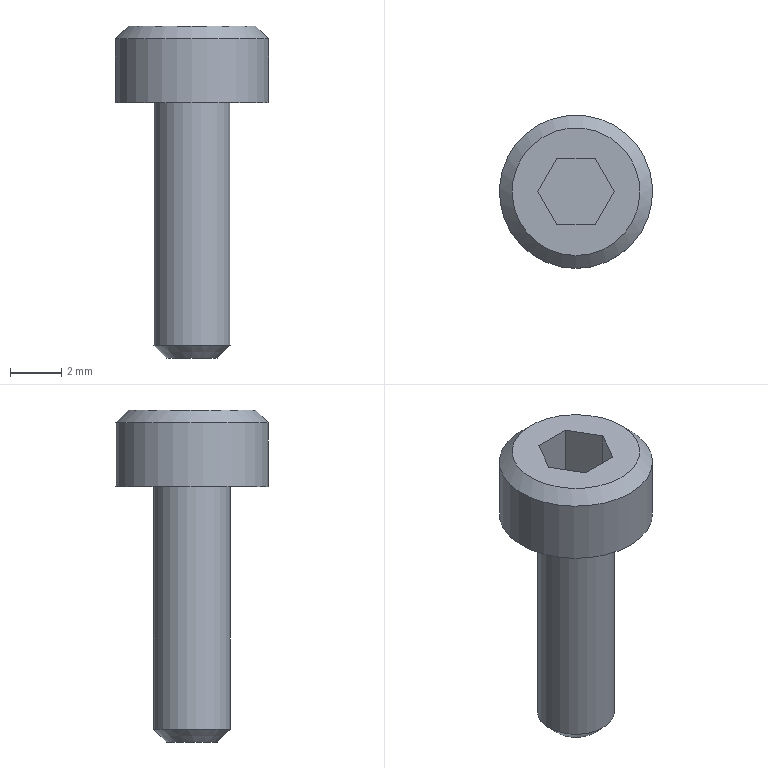Component | NX | SCREW_2 | 1 solid | 14 faces | box 6 x 6 x 13 mm | volume 141 mm3 | plane 10 | cylinder 2 | cone 2 | commonest cylinder face diameters 6 x1 3 x1
STEP:
#1=CARTESIAN_POINT('',(0.,0.,0.));
#2=DIRECTION('',(0.,0.,1.));
#3=DIRECTION('',(1.,0.,0.));
#4=AXIS2_PLACEMENT_3D('',#1,#2,#3);
#5=CARTESIAN_POINT('',(-30.505,120.395,118.114));
#6=VERTEX_POINT('',#5);
#7=CARTESIAN_POINT('',(-30.505,122.895,118.114));
#8=DIRECTION('',(0.,0.,1.));
#9=DIRECTION('',(0.,-1.,0.));
#10=AXIS2_PLACEMENT_3D('',#7,#8,#9);
#11=CIRCLE('',#10,2.5);
#12=CARTESIAN_POINT('',(-30.505,122.895,118.114));
#13=DIRECTION('',(0.,0.,1.));
#14=DIRECTION('',(0.,-1.,0.));
#15=AXIS2_PLACEMENT_3D('',#12,#13,#14);
#16=PLANE('',#15);
#17=CARTESIAN_POINT('',(0.,0.));
#18=DIRECTION('',(1.,0.));
#19=AXIS2_PLACEMENT_2D('',#17,#18);
#20=CIRCLE('',#19,2.5);
#21=(GEOMETRIC_REPRESENTATION_CONTEXT(2)PARAMETRIC_REPRESENTATION_CONTEXT()REPRESENTATION_CONTEXT('',''));
#22=DEFINITIONAL_REPRESENTATION('',(#20),#21);
#23=PCURVE('',#16,#22);
#24=CARTESIAN_POINT('',(-30.505,122.895,118.114));
#25=DIRECTION('',(0.,-0.,-1.));
#26=DIRECTION('',(0.,1.,-0.));
#27=AXIS2_PLACEMENT_3D('',#24,#25,#26);
#28=CONICAL_SURFACE('',#27,2.5,0.7854);
#29=CARTESIAN_POINT('',(9.425,0.));
#30=DIRECTION('',(-1.,0.));
#31=VECTOR('',#30,1.);
#32=LINE('',#29,#31);
#33=(GEOMETRIC_REPRESENTATION_CONTEXT(2)PARAMETRIC_REPRESENTATION_CONTEXT()REPRESENTATION_CONTEXT('',''));
#34=DEFINITIONAL_REPRESENTATION('',(#32),#33);
#35=PCURVE('',#28,#34);
#36=SURFACE_CURVE('',#11,(#23,#35),.PCURVE_S1.);
#37=EDGE_CURVE('',#6,#6,#36,.T.);
#38=ORIENTED_EDGE('',*,*,#37,.T.);
#39=EDGE_LOOP('',(#38));
#40=FACE_BOUND('',#39,.T.);
#41=CARTESIAN_POINT('',(-31.255,121.595,118.114));
#42=VERTEX_POINT('',#41);
#43=CARTESIAN_POINT('',(-29.755,121.595,118.114));
#44=VERTEX_POINT('',#43);
#45=CARTESIAN_POINT('',(-31.255,121.595,118.114));
#46=DIRECTION('',(1.,-0.,0.));
#47=VECTOR('',#46,1.);
#48=LINE('',#45,#47);
#49=CARTESIAN_POINT('',(1.299,-0.75));
#50=DIRECTION('',(0.,1.));
#51=VECTOR('',#50,1.);
#52=LINE('',#49,#51);
#53=(GEOMETRIC_REPRESENTATION_CONTEXT(2)PARAMETRIC_REPRESENTATION_CONTEXT()REPRESENTATION_CONTEXT('',''));
#54=DEFINITIONAL_REPRESENTATION('',(#52),#53);
#55=PCURVE('',#16,#54);
#56=CARTESIAN_POINT('',(-31.255,121.595,116.114));
#57=DIRECTION('',(-0.,-1.,0.));
#58=DIRECTION('',(-1.,0.,-0.));
#59=AXIS2_PLACEMENT_3D('',#56,#57,#58);
#60=PLANE('',#59);
#61=CARTESIAN_POINT('',(-0.,-2.));
#62=DIRECTION('',(-1.,-0.));
#63=VECTOR('',#62,1.);
#64=LINE('',#61,#63);
#65=(GEOMETRIC_REPRESENTATION_CONTEXT(2)PARAMETRIC_REPRESENTATION_CONTEXT()REPRESENTATION_CONTEXT('',''));
#66=DEFINITIONAL_REPRESENTATION('',(#64),#65);
#67=PCURVE('',#60,#66);
#68=SURFACE_CURVE('',#48,(#55,#67),.PCURVE_S1.);
#69=EDGE_CURVE('',#42,#44,#68,.T.);
#70=ORIENTED_EDGE('',*,*,#69,.F.);
#71=CARTESIAN_POINT('',(-32.005,122.895,118.114));
#72=VERTEX_POINT('',#71);
#73=CARTESIAN_POINT('',(-32.005,122.895,118.114));
#74=DIRECTION('',(0.5,-0.866,0.));
#75=VECTOR('',#74,1.);
#76=LINE('',#73,#75);
#77=CARTESIAN_POINT('',(0.,-1.5));
#78=DIRECTION('',(0.866,0.5));
#79=VECTOR('',#78,1.);
#80=LINE('',#77,#79);
#81=(GEOMETRIC_REPRESENTATION_CONTEXT(2)PARAMETRIC_REPRESENTATION_CONTEXT()REPRESENTATION_CONTEXT('',''));
#82=DEFINITIONAL_REPRESENTATION('',(#80),#81);
#83=PCURVE('',#16,#82);
#84=CARTESIAN_POINT('',(-32.005,122.895,116.114));
#85=DIRECTION('',(-0.866,-0.5,0.));
#86=DIRECTION('',(-0.5,0.866,0.));
#87=AXIS2_PLACEMENT_3D('',#84,#85,#86);
#88=PLANE('',#87);
#89=CARTESIAN_POINT('',(0.,-2.));
#90=DIRECTION('',(-1.,-0.));
#91=VECTOR('',#90,1.);
#92=LINE('',#89,#91);
#93=(GEOMETRIC_REPRESENTATION_CONTEXT(2)PARAMETRIC_REPRESENTATION_CONTEXT()REPRESENTATION_CONTEXT('',''));
#94=DEFINITIONAL_REPRESENTATION('',(#92),#93);
#95=PCURVE('',#88,#94);
#96=SURFACE_CURVE('',#76,(#83,#95),.PCURVE_S1.);
#97=EDGE_CURVE('',#72,#42,#96,.T.);
#98=ORIENTED_EDGE('',*,*,#97,.F.);
#99=CARTESIAN_POINT('',(-31.255,124.194,118.114));
#100=VERTEX_POINT('',#99);
#101=CARTESIAN_POINT('',(-31.255,124.194,118.114));
#102=DIRECTION('',(-0.5,-0.866,0.));
#103=VECTOR('',#102,1.);
#104=LINE('',#101,#103);
#105=CARTESIAN_POINT('',(-1.299,-0.75));
#106=DIRECTION('',(0.866,-0.5));
#107=VECTOR('',#106,1.);
#108=LINE('',#105,#107);
#109=(GEOMETRIC_REPRESENTATION_CONTEXT(2)PARAMETRIC_REPRESENTATION_CONTEXT()REPRESENTATION_CONTEXT('',''));
#110=DEFINITIONAL_REPRESENTATION('',(#108),#109);
#111=PCURVE('',#16,#110);
#112=CARTESIAN_POINT('',(-31.255,124.194,116.114));
#113=DIRECTION('',(-0.866,0.5,-0.));
#114=DIRECTION('',(0.5,0.866,0.));
#115=AXIS2_PLACEMENT_3D('',#112,#113,#114);
#116=PLANE('',#115);
#117=CARTESIAN_POINT('',(0.,-2.));
#118=DIRECTION('',(-1.,-0.));
#119=VECTOR('',#118,1.);
#120=LINE('',#117,#119);
#121=(GEOMETRIC_REPRESENTATION_CONTEXT(2)PARAMETRIC_REPRESENTATION_CONTEXT()REPRESENTATION_CONTEXT('',''));
#122=DEFINITIONAL_REPRESENTATION('',(#120),#121);
#123=PCURVE('',#116,#122);
#124=SURFACE_CURVE('',#104,(#111,#123),.PCURVE_S1.);
#125=EDGE_CURVE('',#100,#72,#124,.T.);
#126=ORIENTED_EDGE('',*,*,#125,.F.);
#127=CARTESIAN_POINT('',(-29.755,124.194,118.114));
#128=VERTEX_POINT('',#127);
#129=CARTESIAN_POINT('',(-29.755,124.194,118.114));
#130=DIRECTION('',(-1.,0.,-0.));
#131=VECTOR('',#130,1.);
#132=LINE('',#129,#131);
#133=CARTESIAN_POINT('',(-1.299,0.75));
#134=DIRECTION('',(-0.,-1.));
#135=VECTOR('',#134,1.);
#136=LINE('',#133,#135);
#137=(GEOMETRIC_REPRESENTATION_CONTEXT(2)PARAMETRIC_REPRESENTATION_CONTEXT()REPRESENTATION_CONTEXT('',''));
#138=DEFINITIONAL_REPRESENTATION('',(#136),#137);
#139=PCURVE('',#16,#138);
#140=CARTESIAN_POINT('',(-29.755,124.194,116.114));
#141=DIRECTION('',(0.,1.,-0.));
#142=DIRECTION('',(1.,-0.,0.));
#143=AXIS2_PLACEMENT_3D('',#140,#141,#142);
#144=PLANE('',#143);
#145=CARTESIAN_POINT('',(0.,-2.));
#146=DIRECTION('',(-1.,0.));
#147=VECTOR('',#146,1.);
#148=LINE('',#145,#147);
#149=(GEOMETRIC_REPRESENTATION_CONTEXT(2)PARAMETRIC_REPRESENTATION_CONTEXT()REPRESENTATION_CONTEXT('',''));
#150=DEFINITIONAL_REPRESENTATION('',(#148),#149);
#151=PCURVE('',#144,#150);
#152=SURFACE_CURVE('',#132,(#139,#151),.PCURVE_S1.);
#153=EDGE_CURVE('',#128,#100,#152,.T.);
#154=ORIENTED_EDGE('',*,*,#153,.F.);
#155=CARTESIAN_POINT('',(-29.005,122.895,118.114));
#156=VERTEX_POINT('',#155);
#157=CARTESIAN_POINT('',(-29.005,122.895,118.114));
#158=DIRECTION('',(-0.5,0.866,-0.));
#159=VECTOR('',#158,1.);
#160=LINE('',#157,#159);
#161=CARTESIAN_POINT('',(0.,1.5));
#162=DIRECTION('',(-0.866,-0.5));
#163=VECTOR('',#162,1.);
#164=LINE('',#161,#163);
#165=(GEOMETRIC_REPRESENTATION_CONTEXT(2)PARAMETRIC_REPRESENTATION_CONTEXT()REPRESENTATION_CONTEXT('',''));
#166=DEFINITIONAL_REPRESENTATION('',(#164),#165);
#167=PCURVE('',#16,#166);
#168=CARTESIAN_POINT('',(-29.005,122.895,116.114));
#169=DIRECTION('',(0.866,0.5,-0.));
#170=DIRECTION('',(0.5,-0.866,-0.));
#171=AXIS2_PLACEMENT_3D('',#168,#169,#170);
#172=PLANE('',#171);
#173=CARTESIAN_POINT('',(-0.,-2.));
#174=DIRECTION('',(-1.,0.));
#175=VECTOR('',#174,1.);
#176=LINE('',#173,#175);
#177=(GEOMETRIC_REPRESENTATION_CONTEXT(2)PARAMETRIC_REPRESENTATION_CONTEXT()REPRESENTATION_CONTEXT('',''));
#178=DEFINITIONAL_REPRESENTATION('',(#176),#177);
#179=PCURVE('',#172,#178);
#180=SURFACE_CURVE('',#160,(#167,#179),.PCURVE_S1.);
#181=EDGE_CURVE('',#156,#128,#180,.T.);
#182=ORIENTED_EDGE('',*,*,#181,.F.);
#183=CARTESIAN_POINT('',(-29.755,121.595,118.114));
#184=DIRECTION('',(0.5,0.866,-0.));
#185=VECTOR('',#184,1.);
#186=LINE('',#183,#185);
#187=CARTESIAN_POINT('',(1.299,0.75));
#188=DIRECTION('',(-0.866,0.5));
#189=VECTOR('',#188,1.);
#190=LINE('',#187,#189);
#191=(GEOMETRIC_REPRESENTATION_CONTEXT(2)PARAMETRIC_REPRESENTATION_CONTEXT()REPRESENTATION_CONTEXT('',''));
#192=DEFINITIONAL_REPRESENTATION('',(#190),#191);
#193=PCURVE('',#16,#192);
#194=CARTESIAN_POINT('',(-29.755,121.595,116.114));
#195=DIRECTION('',(0.866,-0.5,0.));
#196=DIRECTION('',(-0.5,-0.866,0.));
#197=AXIS2_PLACEMENT_3D('',#194,#195,#196);
#198=PLANE('',#197);
#199=CARTESIAN_POINT('',(0.,-2.));
#200=DIRECTION('',(-1.,0.));
#201=VECTOR('',#200,1.);
#202=LINE('',#199,#201);
#203=(GEOMETRIC_REPRESENTATION_CONTEXT(2)PARAMETRIC_REPRESENTATION_CONTEXT()REPRESENTATION_CONTEXT('',''));
#204=DEFINITIONAL_REPRESENTATION('',(#202),#203);
#205=PCURVE('',#198,#204);
#206=SURFACE_CURVE('',#186,(#193,#205),.PCURVE_S1.);
#207=EDGE_CURVE('',#44,#156,#206,.T.);
#208=ORIENTED_EDGE('',*,*,#207,.F.);
#209=EDGE_LOOP('',(#70,#98,#126,#154,#182,#208));
#210=FACE_BOUND('',#209,.T.);
#211=ADVANCED_FACE('',(#40,#210),#16,.T.);
#212=CARTESIAN_POINT('',(-30.505,119.895,117.614));
#213=VERTEX_POINT('',#212);
#214=CARTESIAN_POINT('',(-30.505,122.895,117.614));
#215=DIRECTION('',(0.,-0.,-1.));
#216=DIRECTION('',(0.,-1.,0.));
#217=AXIS2_PLACEMENT_3D('',#214,#215,#216);
#218=CIRCLE('',#217,3.);
#219=CARTESIAN_POINT('',(-30.505,122.895,105.114));
#220=DIRECTION('',(0.,0.,1.));
#221=DIRECTION('',(0.,-1.,0.));
#222=AXIS2_PLACEMENT_3D('',#219,#220,#221);
#223=CYLINDRICAL_SURFACE('',#222,3.);
#224=CARTESIAN_POINT('',(6.283,12.5));
#225=DIRECTION('',(-1.,0.));
#226=VECTOR('',#225,1.);
#227=LINE('',#224,#226);
#228=(GEOMETRIC_REPRESENTATION_CONTEXT(2)PARAMETRIC_REPRESENTATION_CONTEXT()REPRESENTATION_CONTEXT('',''));
#229=DEFINITIONAL_REPRESENTATION('',(#227),#228);
#230=PCURVE('',#223,#229);
#231=CARTESIAN_POINT('',(3.142,0.5));
#232=DIRECTION('',(1.,0.));
#233=VECTOR('',#232,1.);
#234=LINE('',#231,#233);
#235=(GEOMETRIC_REPRESENTATION_CONTEXT(2)PARAMETRIC_REPRESENTATION_CONTEXT()REPRESENTATION_CONTEXT('',''));
#236=DEFINITIONAL_REPRESENTATION('',(#234),#235);
#237=PCURVE('',#28,#236);
#238=SURFACE_CURVE('',#218,(#230,#237),.PCURVE_S1.);
#239=EDGE_CURVE('',#213,#213,#238,.T.);
#240=ORIENTED_EDGE('',*,*,#239,.T.);
#241=CARTESIAN_POINT('',(-30.505,119.895,115.114));
#242=VERTEX_POINT('',#241);
#243=CARTESIAN_POINT('',(-30.505,119.895,115.114));
#244=CARTESIAN_POINT('',(-30.505,119.895,117.614));
#245=B_SPLINE_CURVE_WITH_KNOTS('',1,(#243,#244),.UNSPECIFIED.,.F.,.F.,(2,2),(10.,12.5),.PIECEWISE_BEZIER_KNOTS.);
#246=CARTESIAN_POINT('',(0.,0.));
#247=DIRECTION('',(0.,1.));
#248=VECTOR('',#247,1.);
#249=LINE('',#246,#248);
#250=(GEOMETRIC_REPRESENTATION_CONTEXT(2)PARAMETRIC_REPRESENTATION_CONTEXT()REPRESENTATION_CONTEXT('',''));
#251=DEFINITIONAL_REPRESENTATION('',(#249),#250);
#252=PCURVE('',#223,#251);
#253=CARTESIAN_POINT('',(6.283,0.));
#254=DIRECTION('',(0.,1.));
#255=VECTOR('',#254,1.);
#256=LINE('',#253,#255);
#257=(GEOMETRIC_REPRESENTATION_CONTEXT(2)PARAMETRIC_REPRESENTATION_CONTEXT()REPRESENTATION_CONTEXT('',''));
#258=DEFINITIONAL_REPRESENTATION('',(#256),#257);
#259=PCURVE('',#223,#258);
#260=SEAM_CURVE('',#245,(#252,#259),.PCURVE_S1.);
#261=EDGE_CURVE('',#242,#213,#260,.T.);
#262=ORIENTED_EDGE('',*,*,#261,.F.);
#263=CARTESIAN_POINT('',(-30.505,122.895,115.114));
#264=DIRECTION('',(0.,0.,1.));
#265=DIRECTION('',(0.,-1.,0.));
#266=AXIS2_PLACEMENT_3D('',#263,#264,#265);
#267=CIRCLE('',#266,3.);
#268=CARTESIAN_POINT('',(0.,10.));
#269=DIRECTION('',(1.,0.));
#270=VECTOR('',#269,1.);
#271=LINE('',#268,#270);
#272=(GEOMETRIC_REPRESENTATION_CONTEXT(2)PARAMETRIC_REPRESENTATION_CONTEXT()REPRESENTATION_CONTEXT('',''));
#273=DEFINITIONAL_REPRESENTATION('',(#271),#272);
#274=PCURVE('',#223,#273);
#275=CARTESIAN_POINT('',(-30.505,119.895,115.114));
#276=DIRECTION('',(0.,-0.,-1.));
#277=DIRECTION('',(0.,1.,-0.));
#278=AXIS2_PLACEMENT_3D('',#275,#276,#277);
#279=PLANE('',#278);
#280=CARTESIAN_POINT('',(-0.,0.));
#281=CARTESIAN_POINT('',(-0.,5.196));
#282=CARTESIAN_POINT('',(4.5,2.598));
#283=CARTESIAN_POINT('',(9.,0.));
#284=CARTESIAN_POINT('',(4.5,-2.598));
#285=CARTESIAN_POINT('',(-0.,-5.196));
#286=CARTESIAN_POINT('',(-0.,0.));
#287=(BOUNDED_CURVE()B_SPLINE_CURVE(2,(#280,#281,#282,#283,#284,#285,#286),.UNSPECIFIED.,.T.,.F.)B_SPLINE_CURVE_WITH_KNOTS((1,2,2,2,2,1),(-2.094,0.,2.094,4.189,6.283,8.378),.UNSPECIFIED.)CURVE()GEOMETRIC_REPRESENTATION_ITEM()RATIONAL_B_SPLINE_CURVE((1.,0.5,1.,0.5,1.,0.5,1.))REPRESENTATION_ITEM(''));
#288=(GEOMETRIC_REPRESENTATION_CONTEXT(2)PARAMETRIC_REPRESENTATION_CONTEXT()REPRESENTATION_CONTEXT('',''));
#289=DEFINITIONAL_REPRESENTATION('',(#287),#288);
#290=PCURVE('',#279,#289);
#291=SURFACE_CURVE('',#267,(#274,#290),.PCURVE_S1.);
#292=EDGE_CURVE('',#242,#242,#291,.T.);
#293=ORIENTED_EDGE('',*,*,#292,.T.);
#294=ORIENTED_EDGE('',*,*,#261,.T.);
#295=EDGE_LOOP('',(#240,#262,#293,#294));
#296=FACE_BOUND('',#295,.T.);
#297=ADVANCED_FACE('',(#296),#223,.T.);
#298=CARTESIAN_POINT('',(-30.505,121.395,115.114));
#299=VERTEX_POINT('',#298);
#300=CARTESIAN_POINT('',(-30.505,122.895,115.114));
#301=DIRECTION('',(0.,0.,1.));
#302=DIRECTION('',(0.,-1.,0.));
#303=AXIS2_PLACEMENT_3D('',#300,#301,#302);
#304=CIRCLE('',#303,1.5);
#305=CARTESIAN_POINT('',(1.5,0.));
#306=CARTESIAN_POINT('',(1.5,2.598));
#307=CARTESIAN_POINT('',(3.75,1.299));
#308=CARTESIAN_POINT('',(6.,0.));
#309=CARTESIAN_POINT('',(3.75,-1.299));
#310=CARTESIAN_POINT('',(1.5,-2.598));
#311=CARTESIAN_POINT('',(1.5,0.));
#312=(BOUNDED_CURVE()B_SPLINE_CURVE(2,(#305,#306,#307,#308,#309,#310,#311),.UNSPECIFIED.,.T.,.F.)B_SPLINE_CURVE_WITH_KNOTS((1,2,2,2,2,1),(-2.094,0.,2.094,4.189,6.283,8.378),.UNSPECIFIED.)CURVE()GEOMETRIC_REPRESENTATION_ITEM()RATIONAL_B_SPLINE_CURVE((1.,0.5,1.,0.5,1.,0.5,1.))REPRESENTATION_ITEM(''));
#313=(GEOMETRIC_REPRESENTATION_CONTEXT(2)PARAMETRIC_REPRESENTATION_CONTEXT()REPRESENTATION_CONTEXT('',''));
#314=DEFINITIONAL_REPRESENTATION('',(#312),#313);
#315=PCURVE('',#279,#314);
#316=CARTESIAN_POINT('',(-30.505,122.895,105.114));
#317=DIRECTION('',(0.,0.,1.));
#318=DIRECTION('',(0.,-1.,0.));
#319=AXIS2_PLACEMENT_3D('',#316,#317,#318);
#320=CYLINDRICAL_SURFACE('',#319,1.5);
#321=CARTESIAN_POINT('',(0.,10.));
#322=DIRECTION('',(1.,0.));
#323=VECTOR('',#322,1.);
#324=LINE('',#321,#323);
#325=(GEOMETRIC_REPRESENTATION_CONTEXT(2)PARAMETRIC_REPRESENTATION_CONTEXT()REPRESENTATION_CONTEXT('',''));
#326=DEFINITIONAL_REPRESENTATION('',(#324),#325);
#327=PCURVE('',#320,#326);
#328=SURFACE_CURVE('',#304,(#315,#327),.PCURVE_S1.);
#329=EDGE_CURVE('',#299,#299,#328,.T.);
#330=ORIENTED_EDGE('',*,*,#329,.T.);
#331=EDGE_LOOP('',(#330));
#332=FACE_BOUND('',#331,.T.);
#333=ORIENTED_EDGE('',*,*,#292,.F.);
#334=EDGE_LOOP('',(#333));
#335=FACE_BOUND('',#334,.T.);
#336=ADVANCED_FACE('',(#332,#335),#279,.T.);
#337=CARTESIAN_POINT('',(-30.505,124.395,105.614));
#338=VERTEX_POINT('',#337);
#339=CARTESIAN_POINT('',(-30.505,121.395,105.614));
#340=VERTEX_POINT('',#339);
#341=CARTESIAN_POINT('',(-30.505,122.895,105.614));
#342=DIRECTION('',(0.,0.,1.));
#343=DIRECTION('',(0.,1.,-0.));
#344=AXIS2_PLACEMENT_3D('',#341,#342,#343);
#345=CIRCLE('',#344,1.5);
#346=CARTESIAN_POINT('',(3.142,0.5));
#347=DIRECTION('',(1.,0.));
#348=VECTOR('',#347,1.);
#349=LINE('',#346,#348);
#350=(GEOMETRIC_REPRESENTATION_CONTEXT(2)PARAMETRIC_REPRESENTATION_CONTEXT()REPRESENTATION_CONTEXT('',''));
#351=DEFINITIONAL_REPRESENTATION('',(#349),#350);
#352=PCURVE('',#320,#351);
#353=CARTESIAN_POINT('',(-30.505,122.895,105.614));
#354=DIRECTION('',(0.,0.,1.));
#355=DIRECTION('',(0.,-1.,0.));
#356=AXIS2_PLACEMENT_3D('',#353,#354,#355);
#357=CONICAL_SURFACE('',#356,1.5,0.7854);
#358=CARTESIAN_POINT('',(3.142,0.));
#359=DIRECTION('',(1.,0.));
#360=VECTOR('',#359,1.);
#361=LINE('',#358,#360);
#362=(GEOMETRIC_REPRESENTATION_CONTEXT(2)PARAMETRIC_REPRESENTATION_CONTEXT()REPRESENTATION_CONTEXT('',''));
#363=DEFINITIONAL_REPRESENTATION('',(#361),#362);
#364=PCURVE('',#357,#363);
#365=SURFACE_CURVE('',#345,(#352,#364),.PCURVE_S1.);
#366=EDGE_CURVE('',#338,#340,#365,.T.);
#367=ORIENTED_EDGE('',*,*,#366,.T.);
#368=CARTESIAN_POINT('',(-30.505,121.395,105.614));
#369=CARTESIAN_POINT('',(-30.505,121.395,115.114));
#370=B_SPLINE_CURVE_WITH_KNOTS('',1,(#368,#369),.UNSPECIFIED.,.F.,.F.,(2,2),(0.5,10.),.PIECEWISE_BEZIER_KNOTS.);
#371=CARTESIAN_POINT('',(6.283,0.));
#372=DIRECTION('',(0.,1.));
#373=VECTOR('',#372,1.);
#374=LINE('',#371,#373);
#375=(GEOMETRIC_REPRESENTATION_CONTEXT(2)PARAMETRIC_REPRESENTATION_CONTEXT()REPRESENTATION_CONTEXT('',''));
#376=DEFINITIONAL_REPRESENTATION('',(#374),#375);
#377=PCURVE('',#320,#376);
#378=CARTESIAN_POINT('',(0.,0.));
#379=DIRECTION('',(0.,1.));
#380=VECTOR('',#379,1.);
#381=LINE('',#378,#380);
#382=(GEOMETRIC_REPRESENTATION_CONTEXT(2)PARAMETRIC_REPRESENTATION_CONTEXT()REPRESENTATION_CONTEXT('',''));
#383=DEFINITIONAL_REPRESENTATION('',(#381),#382);
#384=PCURVE('',#320,#383);
#385=SEAM_CURVE('',#370,(#377,#384),.PCURVE_S1.);
#386=EDGE_CURVE('',#340,#299,#385,.T.);
#387=ORIENTED_EDGE('',*,*,#386,.T.);
#388=ORIENTED_EDGE('',*,*,#329,.F.);
#389=ORIENTED_EDGE('',*,*,#386,.F.);
#390=CARTESIAN_POINT('',(-30.505,122.895,105.614));
#391=DIRECTION('',(0.,0.,1.));
#392=DIRECTION('',(0.,1.,-0.));
#393=AXIS2_PLACEMENT_3D('',#390,#391,#392);
#394=CIRCLE('',#393,1.5);
#395=CARTESIAN_POINT('',(-3.142,0.5));
#396=DIRECTION('',(1.,0.));
#397=VECTOR('',#396,1.);
#398=LINE('',#395,#397);
#399=(GEOMETRIC_REPRESENTATION_CONTEXT(2)PARAMETRIC_REPRESENTATION_CONTEXT()REPRESENTATION_CONTEXT('',''));
#400=DEFINITIONAL_REPRESENTATION('',(#398),#399);
#401=PCURVE('',#320,#400);
#402=CARTESIAN_POINT('',(3.142,0.));
#403=DIRECTION('',(1.,0.));
#404=VECTOR('',#403,1.);
#405=LINE('',#402,#404);
#406=(GEOMETRIC_REPRESENTATION_CONTEXT(2)PARAMETRIC_REPRESENTATION_CONTEXT()REPRESENTATION_CONTEXT('',''));
#407=DEFINITIONAL_REPRESENTATION('',(#405),#406);
#408=PCURVE('',#357,#407);
#409=SURFACE_CURVE('',#394,(#401,#408),.PCURVE_S1.);
#410=EDGE_CURVE('',#340,#338,#409,.T.);
#411=ORIENTED_EDGE('',*,*,#410,.T.);
#412=EDGE_LOOP('',(#367,#387,#388,#389,#411));
#413=FACE_BOUND('',#412,.T.);
#414=ADVANCED_FACE('',(#413),#320,.T.);
#415=CARTESIAN_POINT('',(-30.505,123.895,105.114));
#416=VERTEX_POINT('',#415);
#417=CARTESIAN_POINT('',(-30.505,122.895,105.114));
#418=DIRECTION('',(0.,-0.,-1.));
#419=DIRECTION('',(0.,1.,-0.));
#420=AXIS2_PLACEMENT_3D('',#417,#418,#419);
#421=CIRCLE('',#420,1.);
#422=CARTESIAN_POINT('',(-30.505,121.395,105.114));
#423=DIRECTION('',(0.,-0.,-1.));
#424=DIRECTION('',(0.,1.,-0.));
#425=AXIS2_PLACEMENT_3D('',#422,#423,#424);
#426=PLANE('',#425);
#427=CARTESIAN_POINT('',(1.5,0.));
#428=DIRECTION('',(1.,0.));
#429=AXIS2_PLACEMENT_2D('',#427,#428);
#430=CIRCLE('',#429,1.);
#431=(GEOMETRIC_REPRESENTATION_CONTEXT(2)PARAMETRIC_REPRESENTATION_CONTEXT()REPRESENTATION_CONTEXT('',''));
#432=DEFINITIONAL_REPRESENTATION('',(#430),#431);
#433=PCURVE('',#426,#432);
#434=CARTESIAN_POINT('',(9.425,-0.5));
#435=DIRECTION('',(-1.,0.));
#436=VECTOR('',#435,1.);
#437=LINE('',#434,#436);
#438=(GEOMETRIC_REPRESENTATION_CONTEXT(2)PARAMETRIC_REPRESENTATION_CONTEXT()REPRESENTATION_CONTEXT('',''));
#439=DEFINITIONAL_REPRESENTATION('',(#437),#438);
#440=PCURVE('',#357,#439);
#441=SURFACE_CURVE('',#421,(#433,#440),.PCURVE_S1.);
#442=EDGE_CURVE('',#416,#416,#441,.T.);
#443=ORIENTED_EDGE('',*,*,#442,.T.);
#444=EDGE_LOOP('',(#443));
#445=FACE_BOUND('',#444,.T.);
#446=ADVANCED_FACE('',(#445),#426,.T.);
#447=ORIENTED_EDGE('',*,*,#69,.T.);
#448=CARTESIAN_POINT('',(-29.755,121.595,116.114));
#449=VERTEX_POINT('',#448);
#450=CARTESIAN_POINT('',(-29.755,121.595,116.114));
#451=DIRECTION('',(0.,-0.,-1.));
#452=VECTOR('',#451,1.);
#453=LINE('',#450,#452);
#454=CARTESIAN_POINT('',(-1.5,-0.));
#455=DIRECTION('',(-0.,1.));
#456=VECTOR('',#455,1.);
#457=LINE('',#454,#456);
#458=(GEOMETRIC_REPRESENTATION_CONTEXT(2)PARAMETRIC_REPRESENTATION_CONTEXT()REPRESENTATION_CONTEXT('',''));
#459=DEFINITIONAL_REPRESENTATION('',(#457),#458);
#460=PCURVE('',#60,#459);
#461=CARTESIAN_POINT('',(0.,0.));
#462=DIRECTION('',(0.,1.));
#463=VECTOR('',#462,1.);
#464=LINE('',#461,#463);
#465=(GEOMETRIC_REPRESENTATION_CONTEXT(2)PARAMETRIC_REPRESENTATION_CONTEXT()REPRESENTATION_CONTEXT('',''));
#466=DEFINITIONAL_REPRESENTATION('',(#464),#465);
#467=PCURVE('',#198,#466);
#468=SURFACE_CURVE('',#453,(#460,#467),.PCURVE_S1.);
#469=EDGE_CURVE('',#44,#449,#468,.T.);
#470=ORIENTED_EDGE('',*,*,#469,.T.);
#471=CARTESIAN_POINT('',(-31.255,121.595,116.114));
#472=VERTEX_POINT('',#471);
#473=CARTESIAN_POINT('',(-31.255,121.595,116.114));
#474=DIRECTION('',(-1.,0.,-0.));
#475=VECTOR('',#474,1.);
#476=LINE('',#473,#475);
#477=CARTESIAN_POINT('',(0.,0.));
#478=DIRECTION('',(1.,0.));
#479=VECTOR('',#478,1.);
#480=LINE('',#477,#479);
#481=(GEOMETRIC_REPRESENTATION_CONTEXT(2)PARAMETRIC_REPRESENTATION_CONTEXT()REPRESENTATION_CONTEXT('',''));
#482=DEFINITIONAL_REPRESENTATION('',(#480),#481);
#483=PCURVE('',#60,#482);
#484=CARTESIAN_POINT('',(-30.505,122.895,116.114));
#485=DIRECTION('',(-0.,0.,1.));
#486=DIRECTION('',(0.,-1.,0.));
#487=AXIS2_PLACEMENT_3D('',#484,#485,#486);
#488=PLANE('',#487);
#489=CARTESIAN_POINT('',(1.299,-0.75));
#490=DIRECTION('',(-0.,-1.));
#491=VECTOR('',#490,1.);
#492=LINE('',#489,#491);
#493=(GEOMETRIC_REPRESENTATION_CONTEXT(2)PARAMETRIC_REPRESENTATION_CONTEXT()REPRESENTATION_CONTEXT('',''));
#494=DEFINITIONAL_REPRESENTATION('',(#492),#493);
#495=PCURVE('',#488,#494);
#496=SURFACE_CURVE('',#476,(#483,#495),.PCURVE_S1.);
#497=EDGE_CURVE('',#449,#472,#496,.T.);
#498=ORIENTED_EDGE('',*,*,#497,.T.);
#499=CARTESIAN_POINT('',(-31.255,121.595,116.114));
#500=DIRECTION('',(0.,-0.,-1.));
#501=VECTOR('',#500,1.);
#502=LINE('',#499,#501);
#503=CARTESIAN_POINT('',(0.,0.));
#504=DIRECTION('',(-0.,1.));
#505=VECTOR('',#504,1.);
#506=LINE('',#503,#505);
#507=(GEOMETRIC_REPRESENTATION_CONTEXT(2)PARAMETRIC_REPRESENTATION_CONTEXT()REPRESENTATION_CONTEXT('',''));
#508=DEFINITIONAL_REPRESENTATION('',(#506),#507);
#509=PCURVE('',#60,#508);
#510=CARTESIAN_POINT('',(-1.5,0.));
#511=DIRECTION('',(-0.,1.));
#512=VECTOR('',#511,1.);
#513=LINE('',#510,#512);
#514=(GEOMETRIC_REPRESENTATION_CONTEXT(2)PARAMETRIC_REPRESENTATION_CONTEXT()REPRESENTATION_CONTEXT('',''));
#515=DEFINITIONAL_REPRESENTATION('',(#513),#514);
#516=PCURVE('',#88,#515);
#517=SURFACE_CURVE('',#502,(#509,#516),.PCURVE_S1.);
#518=EDGE_CURVE('',#42,#472,#517,.T.);
#519=ORIENTED_EDGE('',*,*,#518,.F.);
#520=EDGE_LOOP('',(#447,#470,#498,#519));
#521=FACE_BOUND('',#520,.T.);
#522=ADVANCED_FACE('',(#521),#60,.F.);
#523=ORIENTED_EDGE('',*,*,#207,.T.);
#524=CARTESIAN_POINT('',(-29.005,122.895,116.114));
#525=VERTEX_POINT('',#524);
#526=CARTESIAN_POINT('',(-29.005,122.895,116.114));
#527=DIRECTION('',(0.,-0.,-1.));
#528=VECTOR('',#527,1.);
#529=LINE('',#526,#528);
#530=CARTESIAN_POINT('',(-1.5,0.));
#531=DIRECTION('',(0.,1.));
#532=VECTOR('',#531,1.);
#533=LINE('',#530,#532);
#534=(GEOMETRIC_REPRESENTATION_CONTEXT(2)PARAMETRIC_REPRESENTATION_CONTEXT()REPRESENTATION_CONTEXT('',''));
#535=DEFINITIONAL_REPRESENTATION('',(#533),#534);
#536=PCURVE('',#198,#535);
#537=CARTESIAN_POINT('',(0.,0.));
#538=DIRECTION('',(0.,1.));
#539=VECTOR('',#538,1.);
#540=LINE('',#537,#539);
#541=(GEOMETRIC_REPRESENTATION_CONTEXT(2)PARAMETRIC_REPRESENTATION_CONTEXT()REPRESENTATION_CONTEXT('',''));
#542=DEFINITIONAL_REPRESENTATION('',(#540),#541);
#543=PCURVE('',#172,#542);
#544=SURFACE_CURVE('',#529,(#536,#543),.PCURVE_S1.);
#545=EDGE_CURVE('',#156,#525,#544,.T.);
#546=ORIENTED_EDGE('',*,*,#545,.T.);
#547=CARTESIAN_POINT('',(-29.755,121.595,116.114));
#548=DIRECTION('',(-0.5,-0.866,0.));
#549=VECTOR('',#548,1.);
#550=LINE('',#547,#549);
#551=CARTESIAN_POINT('',(0.,0.));
#552=DIRECTION('',(1.,-0.));
#553=VECTOR('',#552,1.);
#554=LINE('',#551,#553);
#555=(GEOMETRIC_REPRESENTATION_CONTEXT(2)PARAMETRIC_REPRESENTATION_CONTEXT()REPRESENTATION_CONTEXT('',''));
#556=DEFINITIONAL_REPRESENTATION('',(#554),#555);
#557=PCURVE('',#198,#556);
#558=CARTESIAN_POINT('',(1.299,0.75));
#559=DIRECTION('',(0.866,-0.5));
#560=VECTOR('',#559,1.);
#561=LINE('',#558,#560);
#562=(GEOMETRIC_REPRESENTATION_CONTEXT(2)PARAMETRIC_REPRESENTATION_CONTEXT()REPRESENTATION_CONTEXT('',''));
#563=DEFINITIONAL_REPRESENTATION('',(#561),#562);
#564=PCURVE('',#488,#563);
#565=SURFACE_CURVE('',#550,(#557,#564),.PCURVE_S1.);
#566=EDGE_CURVE('',#525,#449,#565,.T.);
#567=ORIENTED_EDGE('',*,*,#566,.T.);
#568=ORIENTED_EDGE('',*,*,#469,.F.);
#569=EDGE_LOOP('',(#523,#546,#567,#568));
#570=FACE_BOUND('',#569,.T.);
#571=ADVANCED_FACE('',(#570),#198,.F.);
#572=ORIENTED_EDGE('',*,*,#181,.T.);
#573=CARTESIAN_POINT('',(-29.755,124.194,116.114));
#574=VERTEX_POINT('',#573);
#575=CARTESIAN_POINT('',(-29.755,124.194,116.114));
#576=DIRECTION('',(0.,-0.,-1.));
#577=VECTOR('',#576,1.);
#578=LINE('',#575,#577);
#579=CARTESIAN_POINT('',(-1.5,0.));
#580=DIRECTION('',(0.,1.));
#581=VECTOR('',#580,1.);
#582=LINE('',#579,#581);
#583=(GEOMETRIC_REPRESENTATION_CONTEXT(2)PARAMETRIC_REPRESENTATION_CONTEXT()REPRESENTATION_CONTEXT('',''));
#584=DEFINITIONAL_REPRESENTATION('',(#582),#583);
#585=PCURVE('',#172,#584);
#586=CARTESIAN_POINT('',(0.,0.));
#587=DIRECTION('',(0.,1.));
#588=VECTOR('',#587,1.);
#589=LINE('',#586,#588);
#590=(GEOMETRIC_REPRESENTATION_CONTEXT(2)PARAMETRIC_REPRESENTATION_CONTEXT()REPRESENTATION_CONTEXT('',''));
#591=DEFINITIONAL_REPRESENTATION('',(#589),#590);
#592=PCURVE('',#144,#591);
#593=SURFACE_CURVE('',#578,(#585,#592),.PCURVE_S1.);
#594=EDGE_CURVE('',#128,#574,#593,.T.);
#595=ORIENTED_EDGE('',*,*,#594,.T.);
#596=CARTESIAN_POINT('',(-29.005,122.895,116.114));
#597=DIRECTION('',(0.5,-0.866,0.));
#598=VECTOR('',#597,1.);
#599=LINE('',#596,#598);
#600=CARTESIAN_POINT('',(0.,0.));
#601=DIRECTION('',(1.,-0.));
#602=VECTOR('',#601,1.);
#603=LINE('',#600,#602);
#604=(GEOMETRIC_REPRESENTATION_CONTEXT(2)PARAMETRIC_REPRESENTATION_CONTEXT()REPRESENTATION_CONTEXT('',''));
#605=DEFINITIONAL_REPRESENTATION('',(#603),#604);
#606=PCURVE('',#172,#605);
#607=CARTESIAN_POINT('',(0.,1.5));
#608=DIRECTION('',(0.866,0.5));
#609=VECTOR('',#608,1.);
#610=LINE('',#607,#609);
#611=(GEOMETRIC_REPRESENTATION_CONTEXT(2)PARAMETRIC_REPRESENTATION_CONTEXT()REPRESENTATION_CONTEXT('',''));
#612=DEFINITIONAL_REPRESENTATION('',(#610),#611);
#613=PCURVE('',#488,#612);
#614=SURFACE_CURVE('',#599,(#606,#613),.PCURVE_S1.);
#615=EDGE_CURVE('',#574,#525,#614,.T.);
#616=ORIENTED_EDGE('',*,*,#615,.T.);
#617=ORIENTED_EDGE('',*,*,#545,.F.);
#618=EDGE_LOOP('',(#572,#595,#616,#617));
#619=FACE_BOUND('',#618,.T.);
#620=ADVANCED_FACE('',(#619),#172,.F.);
#621=ORIENTED_EDGE('',*,*,#153,.T.);
#622=CARTESIAN_POINT('',(-31.255,124.194,116.114));
#623=VERTEX_POINT('',#622);
#624=CARTESIAN_POINT('',(-31.255,124.194,116.114));
#625=DIRECTION('',(0.,-0.,-1.));
#626=VECTOR('',#625,1.);
#627=LINE('',#624,#626);
#628=CARTESIAN_POINT('',(-1.5,0.));
#629=DIRECTION('',(0.,1.));
#630=VECTOR('',#629,1.);
#631=LINE('',#628,#630);
#632=(GEOMETRIC_REPRESENTATION_CONTEXT(2)PARAMETRIC_REPRESENTATION_CONTEXT()REPRESENTATION_CONTEXT('',''));
#633=DEFINITIONAL_REPRESENTATION('',(#631),#632);
#634=PCURVE('',#144,#633);
#635=CARTESIAN_POINT('',(0.,0.));
#636=DIRECTION('',(-0.,1.));
#637=VECTOR('',#636,1.);
#638=LINE('',#635,#637);
#639=(GEOMETRIC_REPRESENTATION_CONTEXT(2)PARAMETRIC_REPRESENTATION_CONTEXT()REPRESENTATION_CONTEXT('',''));
#640=DEFINITIONAL_REPRESENTATION('',(#638),#639);
#641=PCURVE('',#116,#640);
#642=SURFACE_CURVE('',#627,(#634,#641),.PCURVE_S1.);
#643=EDGE_CURVE('',#100,#623,#642,.T.);
#644=ORIENTED_EDGE('',*,*,#643,.T.);
#645=CARTESIAN_POINT('',(-29.755,124.194,116.114));
#646=DIRECTION('',(1.,-0.,0.));
#647=VECTOR('',#646,1.);
#648=LINE('',#645,#647);
#649=CARTESIAN_POINT('',(0.,0.));
#650=DIRECTION('',(1.,-0.));
#651=VECTOR('',#650,1.);
#652=LINE('',#649,#651);
#653=(GEOMETRIC_REPRESENTATION_CONTEXT(2)PARAMETRIC_REPRESENTATION_CONTEXT()REPRESENTATION_CONTEXT('',''));
#654=DEFINITIONAL_REPRESENTATION('',(#652),#653);
#655=PCURVE('',#144,#654);
#656=CARTESIAN_POINT('',(-1.299,0.75));
#657=DIRECTION('',(0.,1.));
#658=VECTOR('',#657,1.);
#659=LINE('',#656,#658);
#660=(GEOMETRIC_REPRESENTATION_CONTEXT(2)PARAMETRIC_REPRESENTATION_CONTEXT()REPRESENTATION_CONTEXT('',''));
#661=DEFINITIONAL_REPRESENTATION('',(#659),#660);
#662=PCURVE('',#488,#661);
#663=SURFACE_CURVE('',#648,(#655,#662),.PCURVE_S1.);
#664=EDGE_CURVE('',#623,#574,#663,.T.);
#665=ORIENTED_EDGE('',*,*,#664,.T.);
#666=ORIENTED_EDGE('',*,*,#594,.F.);
#667=EDGE_LOOP('',(#621,#644,#665,#666));
#668=FACE_BOUND('',#667,.T.);
#669=ADVANCED_FACE('',(#668),#144,.F.);
#670=ORIENTED_EDGE('',*,*,#125,.T.);
#671=CARTESIAN_POINT('',(-32.005,122.895,116.114));
#672=VERTEX_POINT('',#671);
#673=CARTESIAN_POINT('',(-32.005,122.895,116.114));
#674=DIRECTION('',(0.,-0.,-1.));
#675=VECTOR('',#674,1.);
#676=LINE('',#673,#675);
#677=CARTESIAN_POINT('',(-1.5,0.));
#678=DIRECTION('',(-0.,1.));
#679=VECTOR('',#678,1.);
#680=LINE('',#677,#679);
#681=(GEOMETRIC_REPRESENTATION_CONTEXT(2)PARAMETRIC_REPRESENTATION_CONTEXT()REPRESENTATION_CONTEXT('',''));
#682=DEFINITIONAL_REPRESENTATION('',(#680),#681);
#683=PCURVE('',#116,#682);
#684=CARTESIAN_POINT('',(0.,0.));
#685=DIRECTION('',(-0.,1.));
#686=VECTOR('',#685,1.);
#687=LINE('',#684,#686);
#688=(GEOMETRIC_REPRESENTATION_CONTEXT(2)PARAMETRIC_REPRESENTATION_CONTEXT()REPRESENTATION_CONTEXT('',''));
#689=DEFINITIONAL_REPRESENTATION('',(#687),#688);
#690=PCURVE('',#88,#689);
#691=SURFACE_CURVE('',#676,(#683,#690),.PCURVE_S1.);
#692=EDGE_CURVE('',#72,#672,#691,.T.);
#693=ORIENTED_EDGE('',*,*,#692,.T.);
#694=CARTESIAN_POINT('',(-31.255,124.194,116.114));
#695=DIRECTION('',(0.5,0.866,-0.));
#696=VECTOR('',#695,1.);
#697=LINE('',#694,#696);
#698=CARTESIAN_POINT('',(0.,0.));
#699=DIRECTION('',(1.,0.));
#700=VECTOR('',#699,1.);
#701=LINE('',#698,#700);
#702=(GEOMETRIC_REPRESENTATION_CONTEXT(2)PARAMETRIC_REPRESENTATION_CONTEXT()REPRESENTATION_CONTEXT('',''));
#703=DEFINITIONAL_REPRESENTATION('',(#701),#702);
#704=PCURVE('',#116,#703);
#705=CARTESIAN_POINT('',(-1.299,-0.75));
#706=DIRECTION('',(-0.866,0.5));
#707=VECTOR('',#706,1.);
#708=LINE('',#705,#707);
#709=(GEOMETRIC_REPRESENTATION_CONTEXT(2)PARAMETRIC_REPRESENTATION_CONTEXT()REPRESENTATION_CONTEXT('',''));
#710=DEFINITIONAL_REPRESENTATION('',(#708),#709);
#711=PCURVE('',#488,#710);
#712=SURFACE_CURVE('',#697,(#704,#711),.PCURVE_S1.);
#713=EDGE_CURVE('',#672,#623,#712,.T.);
#714=ORIENTED_EDGE('',*,*,#713,.T.);
#715=ORIENTED_EDGE('',*,*,#643,.F.);
#716=EDGE_LOOP('',(#670,#693,#714,#715));
#717=FACE_BOUND('',#716,.T.);
#718=ADVANCED_FACE('',(#717),#116,.F.);
#719=ORIENTED_EDGE('',*,*,#97,.T.);
#720=ORIENTED_EDGE('',*,*,#518,.T.);
#721=CARTESIAN_POINT('',(-32.005,122.895,116.114));
#722=DIRECTION('',(-0.5,0.866,-0.));
#723=VECTOR('',#722,1.);
#724=LINE('',#721,#723);
#725=CARTESIAN_POINT('',(0.,0.));
#726=DIRECTION('',(1.,0.));
#727=VECTOR('',#726,1.);
#728=LINE('',#725,#727);
#729=(GEOMETRIC_REPRESENTATION_CONTEXT(2)PARAMETRIC_REPRESENTATION_CONTEXT()REPRESENTATION_CONTEXT('',''));
#730=DEFINITIONAL_REPRESENTATION('',(#728),#729);
#731=PCURVE('',#88,#730);
#732=CARTESIAN_POINT('',(-0.,-1.5));
#733=DIRECTION('',(-0.866,-0.5));
#734=VECTOR('',#733,1.);
#735=LINE('',#732,#734);
#736=(GEOMETRIC_REPRESENTATION_CONTEXT(2)PARAMETRIC_REPRESENTATION_CONTEXT()REPRESENTATION_CONTEXT('',''));
#737=DEFINITIONAL_REPRESENTATION('',(#735),#736);
#738=PCURVE('',#488,#737);
#739=SURFACE_CURVE('',#724,(#731,#738),.PCURVE_S1.);
#740=EDGE_CURVE('',#472,#672,#739,.T.);
#741=ORIENTED_EDGE('',*,*,#740,.T.);
#742=ORIENTED_EDGE('',*,*,#692,.F.);
#743=EDGE_LOOP('',(#719,#720,#741,#742));
#744=FACE_BOUND('',#743,.T.);
#745=ADVANCED_FACE('',(#744),#88,.F.);
#746=ORIENTED_EDGE('',*,*,#497,.F.);
#747=ORIENTED_EDGE('',*,*,#566,.F.);
#748=ORIENTED_EDGE('',*,*,#615,.F.);
#749=ORIENTED_EDGE('',*,*,#664,.F.);
#750=ORIENTED_EDGE('',*,*,#713,.F.);
#751=ORIENTED_EDGE('',*,*,#740,.F.);
#752=EDGE_LOOP('',(#746,#747,#748,#749,#750,#751));
#753=FACE_BOUND('',#752,.T.);
#754=ADVANCED_FACE('',(#753),#488,.T.);
#755=ORIENTED_EDGE('',*,*,#239,.F.);
#756=CARTESIAN_POINT('',(-30.505,120.395,118.114));
#757=CARTESIAN_POINT('',(-30.505,119.895,117.614));
#758=B_SPLINE_CURVE_WITH_KNOTS('',1,(#756,#757),.UNSPECIFIED.,.F.,.F.,(2,2),(0.,0.7071),.PIECEWISE_BEZIER_KNOTS.);
#759=CARTESIAN_POINT('',(3.142,0.));
#760=DIRECTION('',(0.,1.));
#761=VECTOR('',#760,1.);
#762=LINE('',#759,#761);
#763=(GEOMETRIC_REPRESENTATION_CONTEXT(2)PARAMETRIC_REPRESENTATION_CONTEXT()REPRESENTATION_CONTEXT('',''));
#764=DEFINITIONAL_REPRESENTATION('',(#762),#763);
#765=PCURVE('',#28,#764);
#766=CARTESIAN_POINT('',(9.425,0.));
#767=DIRECTION('',(0.,1.));
#768=VECTOR('',#767,1.);
#769=LINE('',#766,#768);
#770=(GEOMETRIC_REPRESENTATION_CONTEXT(2)PARAMETRIC_REPRESENTATION_CONTEXT()REPRESENTATION_CONTEXT('',''));
#771=DEFINITIONAL_REPRESENTATION('',(#769),#770);
#772=PCURVE('',#28,#771);
#773=SEAM_CURVE('',#758,(#765,#772),.PCURVE_S1.);
#774=EDGE_CURVE('',#6,#213,#773,.T.);
#775=ORIENTED_EDGE('',*,*,#774,.F.);
#776=ORIENTED_EDGE('',*,*,#37,.F.);
#777=ORIENTED_EDGE('',*,*,#774,.T.);
#778=EDGE_LOOP('',(#755,#775,#776,#777));
#779=FACE_BOUND('',#778,.T.);
#780=ADVANCED_FACE('',(#779),#28,.T.);
#781=ORIENTED_EDGE('',*,*,#442,.F.);
#782=CARTESIAN_POINT('',(-30.505,123.895,105.114));
#783=CARTESIAN_POINT('',(-30.505,124.395,105.614));
#784=B_SPLINE_CURVE_WITH_KNOTS('',1,(#782,#783),.UNSPECIFIED.,.F.,.F.,(2,2),(-0.7071,0.),.PIECEWISE_BEZIER_KNOTS.);
#785=CARTESIAN_POINT('',(9.425,0.));
#786=DIRECTION('',(0.,1.));
#787=VECTOR('',#786,1.);
#788=LINE('',#785,#787);
#789=(GEOMETRIC_REPRESENTATION_CONTEXT(2)PARAMETRIC_REPRESENTATION_CONTEXT()REPRESENTATION_CONTEXT('',''));
#790=DEFINITIONAL_REPRESENTATION('',(#788),#789);
#791=PCURVE('',#357,#790);
#792=CARTESIAN_POINT('',(3.142,0.));
#793=DIRECTION('',(0.,1.));
#794=VECTOR('',#793,1.);
#795=LINE('',#792,#794);
#796=(GEOMETRIC_REPRESENTATION_CONTEXT(2)PARAMETRIC_REPRESENTATION_CONTEXT()REPRESENTATION_CONTEXT('',''));
#797=DEFINITIONAL_REPRESENTATION('',(#795),#796);
#798=PCURVE('',#357,#797);
#799=SEAM_CURVE('',#784,(#791,#798),.PCURVE_S1.);
#800=EDGE_CURVE('',#416,#338,#799,.T.);
#801=ORIENTED_EDGE('',*,*,#800,.T.);
#802=ORIENTED_EDGE('',*,*,#410,.F.);
#803=ORIENTED_EDGE('',*,*,#366,.F.);
#804=ORIENTED_EDGE('',*,*,#800,.F.);
#805=EDGE_LOOP('',(#781,#801,#802,#803,#804));
#806=FACE_BOUND('',#805,.T.);
#807=ADVANCED_FACE('',(#806),#357,.T.);
#808=CLOSED_SHELL('',(#211,#297,#336,#414,#446,#522,#571,#620,#669,#718,#745,#754,#780,#807));
#809=MANIFOLD_SOLID_BREP('',#808);
#810=(LENGTH_UNIT()NAMED_UNIT(*)SI_UNIT(.MILLI.,.METRE.));
#811=UNCERTAINTY_MEASURE_WITH_UNIT(LENGTH_MEASURE(0.000002),#810,'','');
#812=(NAMED_UNIT(*)PLANE_ANGLE_UNIT()SI_UNIT($,.RADIAN.));
#813=(NAMED_UNIT(*)SI_UNIT($,.STERADIAN.)SOLID_ANGLE_UNIT());
#814=(GEOMETRIC_REPRESENTATION_CONTEXT(3)GLOBAL_UNCERTAINTY_ASSIGNED_CONTEXT((#811))GLOBAL_UNIT_ASSIGNED_CONTEXT((#810,#812,#813))REPRESENTATION_CONTEXT('',''));
#815=ADVANCED_BREP_SHAPE_REPRESENTATION('',(#4,#809),#814);